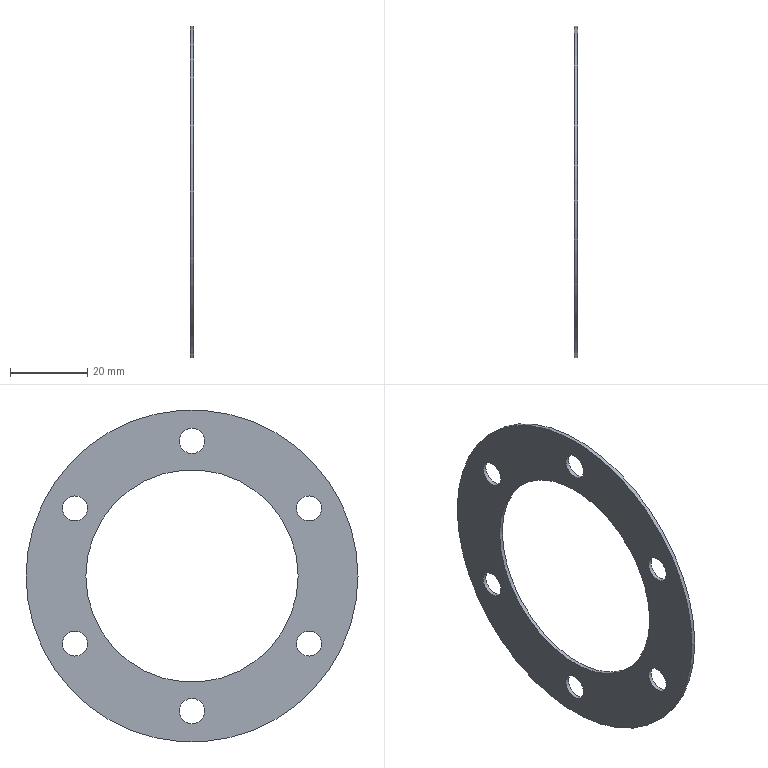Component | NX | XIAODIANPIAN_2 | 1 solid | 10 faces | box 1 x 86 x 86 mm | volume 3234 mm3 | cylinder 8 | plane 2 | commonest cylinder face diameters 6.5 x6 86 x1 55 x1
STEP:
#1=CARTESIAN_POINT('',(0.,0.,0.));
#2=DIRECTION('',(0.,0.,1.));
#3=DIRECTION('',(1.,0.,0.));
#4=AXIS2_PLACEMENT_3D('',#1,#2,#3);
#5=CARTESIAN_POINT('',(-111.,44.5,-88.));
#6=VERTEX_POINT('',#5);
#7=CARTESIAN_POINT('',(-111.,87.5,-88.));
#8=DIRECTION('',(-1.,0.,0.));
#9=DIRECTION('',(0.,-1.,0.));
#10=AXIS2_PLACEMENT_3D('',#7,#8,#9);
#11=CIRCLE('',#10,43.);
#12=CARTESIAN_POINT('',(-111.,87.5,-88.));
#13=DIRECTION('',(1.,0.,0.));
#14=DIRECTION('',(0.,0.,1.));
#15=AXIS2_PLACEMENT_3D('',#12,#13,#14);
#16=CYLINDRICAL_SURFACE('',#15,43.);
#17=CARTESIAN_POINT('',(7.854,0.));
#18=DIRECTION('',(-1.,0.));
#19=VECTOR('',#18,1.);
#20=LINE('',#17,#19);
#21=(GEOMETRIC_REPRESENTATION_CONTEXT(2)PARAMETRIC_REPRESENTATION_CONTEXT()REPRESENTATION_CONTEXT('',''));
#22=DEFINITIONAL_REPRESENTATION('',(#20),#21);
#23=PCURVE('',#16,#22);
#24=CARTESIAN_POINT('',(-111.,87.5,-88.));
#25=DIRECTION('',(-1.,0.,0.));
#26=DIRECTION('',(0.,0.,-1.));
#27=AXIS2_PLACEMENT_3D('',#24,#25,#26);
#28=PLANE('',#27);
#29=CARTESIAN_POINT('',(0.,0.));
#30=DIRECTION('',(0.,1.));
#31=AXIS2_PLACEMENT_2D('',#29,#30);
#32=CIRCLE('',#31,43.);
#33=(GEOMETRIC_REPRESENTATION_CONTEXT(2)PARAMETRIC_REPRESENTATION_CONTEXT()REPRESENTATION_CONTEXT('',''));
#34=DEFINITIONAL_REPRESENTATION('',(#32),#33);
#35=PCURVE('',#28,#34);
#36=SURFACE_CURVE('',#11,(#23,#35),.PCURVE_S1.);
#37=EDGE_CURVE('',#6,#6,#36,.T.);
#38=ORIENTED_EDGE('',*,*,#37,.F.);
#39=CARTESIAN_POINT('',(-110.,44.5,-88.));
#40=VERTEX_POINT('',#39);
#41=CARTESIAN_POINT('',(-111.,44.5,-88.));
#42=CARTESIAN_POINT('',(-110.,44.5,-88.));
#43=B_SPLINE_CURVE_WITH_KNOTS('',1,(#41,#42),.UNSPECIFIED.,.F.,.F.,(2,2),(0.,1.),.PIECEWISE_BEZIER_KNOTS.);
#44=CARTESIAN_POINT('',(7.854,0.));
#45=DIRECTION('',(0.,1.));
#46=VECTOR('',#45,1.);
#47=LINE('',#44,#46);
#48=(GEOMETRIC_REPRESENTATION_CONTEXT(2)PARAMETRIC_REPRESENTATION_CONTEXT()REPRESENTATION_CONTEXT('',''));
#49=DEFINITIONAL_REPRESENTATION('',(#47),#48);
#50=PCURVE('',#16,#49);
#51=CARTESIAN_POINT('',(1.571,0.));
#52=DIRECTION('',(0.,1.));
#53=VECTOR('',#52,1.);
#54=LINE('',#51,#53);
#55=(GEOMETRIC_REPRESENTATION_CONTEXT(2)PARAMETRIC_REPRESENTATION_CONTEXT()REPRESENTATION_CONTEXT('',''));
#56=DEFINITIONAL_REPRESENTATION('',(#54),#55);
#57=PCURVE('',#16,#56);
#58=SEAM_CURVE('',#43,(#50,#57),.PCURVE_S1.);
#59=EDGE_CURVE('',#6,#40,#58,.T.);
#60=ORIENTED_EDGE('',*,*,#59,.T.);
#61=CARTESIAN_POINT('',(-110.,87.5,-88.));
#62=DIRECTION('',(-1.,0.,0.));
#63=DIRECTION('',(0.,-1.,0.));
#64=AXIS2_PLACEMENT_3D('',#61,#62,#63);
#65=CIRCLE('',#64,43.);
#66=CARTESIAN_POINT('',(7.854,1.));
#67=DIRECTION('',(-1.,0.));
#68=VECTOR('',#67,1.);
#69=LINE('',#66,#68);
#70=(GEOMETRIC_REPRESENTATION_CONTEXT(2)PARAMETRIC_REPRESENTATION_CONTEXT()REPRESENTATION_CONTEXT('',''));
#71=DEFINITIONAL_REPRESENTATION('',(#69),#70);
#72=PCURVE('',#16,#71);
#73=CARTESIAN_POINT('',(-110.,87.5,-88.));
#74=DIRECTION('',(-1.,0.,0.));
#75=DIRECTION('',(0.,0.,-1.));
#76=AXIS2_PLACEMENT_3D('',#73,#74,#75);
#77=PLANE('',#76);
#78=CARTESIAN_POINT('',(0.,0.));
#79=DIRECTION('',(0.,1.));
#80=AXIS2_PLACEMENT_2D('',#78,#79);
#81=CIRCLE('',#80,43.);
#82=(GEOMETRIC_REPRESENTATION_CONTEXT(2)PARAMETRIC_REPRESENTATION_CONTEXT()REPRESENTATION_CONTEXT('',''));
#83=DEFINITIONAL_REPRESENTATION('',(#81),#82);
#84=PCURVE('',#77,#83);
#85=SURFACE_CURVE('',#65,(#72,#84),.PCURVE_S1.);
#86=EDGE_CURVE('',#40,#40,#85,.T.);
#87=ORIENTED_EDGE('',*,*,#86,.T.);
#88=ORIENTED_EDGE('',*,*,#59,.F.);
#89=EDGE_LOOP('',(#38,#60,#87,#88));
#90=FACE_BOUND('',#89,.T.);
#91=ADVANCED_FACE('',(#90),#16,.T.);
#92=CARTESIAN_POINT('',(-111.,60.,-88.));
#93=VERTEX_POINT('',#92);
#94=CARTESIAN_POINT('',(-111.,87.5,-88.));
#95=DIRECTION('',(-1.,0.,0.));
#96=DIRECTION('',(0.,-1.,0.));
#97=AXIS2_PLACEMENT_3D('',#94,#95,#96);
#98=CIRCLE('',#97,27.5);
#99=CARTESIAN_POINT('',(-111.,87.5,-88.));
#100=DIRECTION('',(1.,0.,0.));
#101=DIRECTION('',(0.,0.,1.));
#102=AXIS2_PLACEMENT_3D('',#99,#100,#101);
#103=CYLINDRICAL_SURFACE('',#102,27.5);
#104=CARTESIAN_POINT('',(7.854,0.));
#105=DIRECTION('',(-1.,0.));
#106=VECTOR('',#105,1.);
#107=LINE('',#104,#106);
#108=(GEOMETRIC_REPRESENTATION_CONTEXT(2)PARAMETRIC_REPRESENTATION_CONTEXT()REPRESENTATION_CONTEXT('',''));
#109=DEFINITIONAL_REPRESENTATION('',(#107),#108);
#110=PCURVE('',#103,#109);
#111=CARTESIAN_POINT('',(0.,0.));
#112=DIRECTION('',(0.,1.));
#113=AXIS2_PLACEMENT_2D('',#111,#112);
#114=CIRCLE('',#113,27.5);
#115=(GEOMETRIC_REPRESENTATION_CONTEXT(2)PARAMETRIC_REPRESENTATION_CONTEXT()REPRESENTATION_CONTEXT('',''));
#116=DEFINITIONAL_REPRESENTATION('',(#114),#115);
#117=PCURVE('',#28,#116);
#118=SURFACE_CURVE('',#98,(#110,#117),.PCURVE_S1.);
#119=EDGE_CURVE('',#93,#93,#118,.T.);
#120=ORIENTED_EDGE('',*,*,#119,.F.);
#121=CARTESIAN_POINT('',(-110.,60.,-88.));
#122=VERTEX_POINT('',#121);
#123=CARTESIAN_POINT('',(-111.,60.,-88.));
#124=CARTESIAN_POINT('',(-110.,60.,-88.));
#125=B_SPLINE_CURVE_WITH_KNOTS('',1,(#123,#124),.UNSPECIFIED.,.F.,.F.,(2,2),(0.,1.),.PIECEWISE_BEZIER_KNOTS.);
#126=CARTESIAN_POINT('',(7.854,0.));
#127=DIRECTION('',(0.,1.));
#128=VECTOR('',#127,1.);
#129=LINE('',#126,#128);
#130=(GEOMETRIC_REPRESENTATION_CONTEXT(2)PARAMETRIC_REPRESENTATION_CONTEXT()REPRESENTATION_CONTEXT('',''));
#131=DEFINITIONAL_REPRESENTATION('',(#129),#130);
#132=PCURVE('',#103,#131);
#133=CARTESIAN_POINT('',(1.571,0.));
#134=DIRECTION('',(0.,1.));
#135=VECTOR('',#134,1.);
#136=LINE('',#133,#135);
#137=(GEOMETRIC_REPRESENTATION_CONTEXT(2)PARAMETRIC_REPRESENTATION_CONTEXT()REPRESENTATION_CONTEXT('',''));
#138=DEFINITIONAL_REPRESENTATION('',(#136),#137);
#139=PCURVE('',#103,#138);
#140=SEAM_CURVE('',#125,(#132,#139),.PCURVE_S1.);
#141=EDGE_CURVE('',#93,#122,#140,.T.);
#142=ORIENTED_EDGE('',*,*,#141,.T.);
#143=CARTESIAN_POINT('',(-110.,87.5,-88.));
#144=DIRECTION('',(-1.,0.,0.));
#145=DIRECTION('',(0.,-1.,0.));
#146=AXIS2_PLACEMENT_3D('',#143,#144,#145);
#147=CIRCLE('',#146,27.5);
#148=CARTESIAN_POINT('',(7.854,1.));
#149=DIRECTION('',(-1.,0.));
#150=VECTOR('',#149,1.);
#151=LINE('',#148,#150);
#152=(GEOMETRIC_REPRESENTATION_CONTEXT(2)PARAMETRIC_REPRESENTATION_CONTEXT()REPRESENTATION_CONTEXT('',''));
#153=DEFINITIONAL_REPRESENTATION('',(#151),#152);
#154=PCURVE('',#103,#153);
#155=CARTESIAN_POINT('',(0.,0.));
#156=DIRECTION('',(0.,1.));
#157=AXIS2_PLACEMENT_2D('',#155,#156);
#158=CIRCLE('',#157,27.5);
#159=(GEOMETRIC_REPRESENTATION_CONTEXT(2)PARAMETRIC_REPRESENTATION_CONTEXT()REPRESENTATION_CONTEXT('',''));
#160=DEFINITIONAL_REPRESENTATION('',(#158),#159);
#161=PCURVE('',#77,#160);
#162=SURFACE_CURVE('',#147,(#154,#161),.PCURVE_S1.);
#163=EDGE_CURVE('',#122,#122,#162,.T.);
#164=ORIENTED_EDGE('',*,*,#163,.T.);
#165=ORIENTED_EDGE('',*,*,#141,.F.);
#166=EDGE_LOOP('',(#120,#142,#164,#165));
#167=FACE_BOUND('',#166,.F.);
#168=ADVANCED_FACE('',(#167),#103,.F.);
#169=CARTESIAN_POINT('',(-111.,57.189,-73.75));
#170=VERTEX_POINT('',#169);
#171=CARTESIAN_POINT('',(-111.,57.189,-70.5));
#172=DIRECTION('',(-1.,0.,0.));
#173=DIRECTION('',(0.,0.,-1.));
#174=AXIS2_PLACEMENT_3D('',#171,#172,#173);
#175=CIRCLE('',#174,3.25);
#176=CARTESIAN_POINT('',(-17.5,30.311));
#177=DIRECTION('',(1.,0.));
#178=AXIS2_PLACEMENT_2D('',#176,#177);
#179=CIRCLE('',#178,3.25);
#180=(GEOMETRIC_REPRESENTATION_CONTEXT(2)PARAMETRIC_REPRESENTATION_CONTEXT()REPRESENTATION_CONTEXT('',''));
#181=DEFINITIONAL_REPRESENTATION('',(#179),#180);
#182=PCURVE('',#28,#181);
#183=CARTESIAN_POINT('',(-110.,57.189,-70.5));
#184=DIRECTION('',(-1.,0.,0.));
#185=DIRECTION('',(0.,0.,-1.));
#186=AXIS2_PLACEMENT_3D('',#183,#184,#185);
#187=CYLINDRICAL_SURFACE('',#186,3.25);
#188=CARTESIAN_POINT('',(0.,1.));
#189=DIRECTION('',(1.,0.));
#190=VECTOR('',#189,1.);
#191=LINE('',#188,#190);
#192=(GEOMETRIC_REPRESENTATION_CONTEXT(2)PARAMETRIC_REPRESENTATION_CONTEXT()REPRESENTATION_CONTEXT('',''));
#193=DEFINITIONAL_REPRESENTATION('',(#191),#192);
#194=PCURVE('',#187,#193);
#195=SURFACE_CURVE('',#175,(#182,#194),.PCURVE_S1.);
#196=EDGE_CURVE('',#170,#170,#195,.T.);
#197=ORIENTED_EDGE('',*,*,#196,.F.);
#198=EDGE_LOOP('',(#197));
#199=FACE_BOUND('',#198,.T.);
#200=CARTESIAN_POINT('',(-111.,57.189,-108.75));
#201=VERTEX_POINT('',#200);
#202=CARTESIAN_POINT('',(-111.,57.189,-105.5));
#203=DIRECTION('',(-1.,0.,0.));
#204=DIRECTION('',(0.,0.,-1.));
#205=AXIS2_PLACEMENT_3D('',#202,#203,#204);
#206=CIRCLE('',#205,3.25);
#207=CARTESIAN_POINT('',(17.5,30.311));
#208=DIRECTION('',(1.,0.));
#209=AXIS2_PLACEMENT_2D('',#207,#208);
#210=CIRCLE('',#209,3.25);
#211=(GEOMETRIC_REPRESENTATION_CONTEXT(2)PARAMETRIC_REPRESENTATION_CONTEXT()REPRESENTATION_CONTEXT('',''));
#212=DEFINITIONAL_REPRESENTATION('',(#210),#211);
#213=PCURVE('',#28,#212);
#214=CARTESIAN_POINT('',(-110.,57.189,-105.5));
#215=DIRECTION('',(-1.,0.,0.));
#216=DIRECTION('',(0.,0.,-1.));
#217=AXIS2_PLACEMENT_3D('',#214,#215,#216);
#218=CYLINDRICAL_SURFACE('',#217,3.25);
#219=CARTESIAN_POINT('',(0.,1.));
#220=DIRECTION('',(1.,0.));
#221=VECTOR('',#220,1.);
#222=LINE('',#219,#221);
#223=(GEOMETRIC_REPRESENTATION_CONTEXT(2)PARAMETRIC_REPRESENTATION_CONTEXT()REPRESENTATION_CONTEXT('',''));
#224=DEFINITIONAL_REPRESENTATION('',(#222),#223);
#225=PCURVE('',#218,#224);
#226=SURFACE_CURVE('',#206,(#213,#225),.PCURVE_S1.);
#227=EDGE_CURVE('',#201,#201,#226,.T.);
#228=ORIENTED_EDGE('',*,*,#227,.F.);
#229=EDGE_LOOP('',(#228));
#230=FACE_BOUND('',#229,.T.);
#231=CARTESIAN_POINT('',(-111.,87.5,-56.25));
#232=VERTEX_POINT('',#231);
#233=CARTESIAN_POINT('',(-111.,87.5,-53.));
#234=DIRECTION('',(-1.,0.,0.));
#235=DIRECTION('',(0.,0.,-1.));
#236=AXIS2_PLACEMENT_3D('',#233,#234,#235);
#237=CIRCLE('',#236,3.25);
#238=CARTESIAN_POINT('',(-35.,-0.));
#239=DIRECTION('',(1.,0.));
#240=AXIS2_PLACEMENT_2D('',#238,#239);
#241=CIRCLE('',#240,3.25);
#242=(GEOMETRIC_REPRESENTATION_CONTEXT(2)PARAMETRIC_REPRESENTATION_CONTEXT()REPRESENTATION_CONTEXT('',''));
#243=DEFINITIONAL_REPRESENTATION('',(#241),#242);
#244=PCURVE('',#28,#243);
#245=CARTESIAN_POINT('',(-110.,87.5,-53.));
#246=DIRECTION('',(-1.,0.,0.));
#247=DIRECTION('',(0.,0.,-1.));
#248=AXIS2_PLACEMENT_3D('',#245,#246,#247);
#249=CYLINDRICAL_SURFACE('',#248,3.25);
#250=CARTESIAN_POINT('',(0.,1.));
#251=DIRECTION('',(1.,0.));
#252=VECTOR('',#251,1.);
#253=LINE('',#250,#252);
#254=(GEOMETRIC_REPRESENTATION_CONTEXT(2)PARAMETRIC_REPRESENTATION_CONTEXT()REPRESENTATION_CONTEXT('',''));
#255=DEFINITIONAL_REPRESENTATION('',(#253),#254);
#256=PCURVE('',#249,#255);
#257=SURFACE_CURVE('',#237,(#244,#256),.PCURVE_S1.);
#258=EDGE_CURVE('',#232,#232,#257,.T.);
#259=ORIENTED_EDGE('',*,*,#258,.F.);
#260=EDGE_LOOP('',(#259));
#261=FACE_BOUND('',#260,.T.);
#262=CARTESIAN_POINT('',(-111.,87.5,-126.25));
#263=VERTEX_POINT('',#262);
#264=CARTESIAN_POINT('',(-111.,87.5,-123.));
#265=DIRECTION('',(-1.,0.,0.));
#266=DIRECTION('',(0.,0.,-1.));
#267=AXIS2_PLACEMENT_3D('',#264,#265,#266);
#268=CIRCLE('',#267,3.25);
#269=CARTESIAN_POINT('',(35.,0.));
#270=DIRECTION('',(1.,0.));
#271=AXIS2_PLACEMENT_2D('',#269,#270);
#272=CIRCLE('',#271,3.25);
#273=(GEOMETRIC_REPRESENTATION_CONTEXT(2)PARAMETRIC_REPRESENTATION_CONTEXT()REPRESENTATION_CONTEXT('',''));
#274=DEFINITIONAL_REPRESENTATION('',(#272),#273);
#275=PCURVE('',#28,#274);
#276=CARTESIAN_POINT('',(-110.,87.5,-123.));
#277=DIRECTION('',(-1.,0.,0.));
#278=DIRECTION('',(0.,0.,-1.));
#279=AXIS2_PLACEMENT_3D('',#276,#277,#278);
#280=CYLINDRICAL_SURFACE('',#279,3.25);
#281=CARTESIAN_POINT('',(0.,1.));
#282=DIRECTION('',(1.,0.));
#283=VECTOR('',#282,1.);
#284=LINE('',#281,#283);
#285=(GEOMETRIC_REPRESENTATION_CONTEXT(2)PARAMETRIC_REPRESENTATION_CONTEXT()REPRESENTATION_CONTEXT('',''));
#286=DEFINITIONAL_REPRESENTATION('',(#284),#285);
#287=PCURVE('',#280,#286);
#288=SURFACE_CURVE('',#268,(#275,#287),.PCURVE_S1.);
#289=EDGE_CURVE('',#263,#263,#288,.T.);
#290=ORIENTED_EDGE('',*,*,#289,.F.);
#291=EDGE_LOOP('',(#290));
#292=FACE_BOUND('',#291,.T.);
#293=CARTESIAN_POINT('',(-111.,117.811,-73.75));
#294=VERTEX_POINT('',#293);
#295=CARTESIAN_POINT('',(-111.,117.811,-70.5));
#296=DIRECTION('',(-1.,0.,0.));
#297=DIRECTION('',(0.,0.,-1.));
#298=AXIS2_PLACEMENT_3D('',#295,#296,#297);
#299=CIRCLE('',#298,3.25);
#300=CARTESIAN_POINT('',(-17.5,-30.311));
#301=DIRECTION('',(1.,0.));
#302=AXIS2_PLACEMENT_2D('',#300,#301);
#303=CIRCLE('',#302,3.25);
#304=(GEOMETRIC_REPRESENTATION_CONTEXT(2)PARAMETRIC_REPRESENTATION_CONTEXT()REPRESENTATION_CONTEXT('',''));
#305=DEFINITIONAL_REPRESENTATION('',(#303),#304);
#306=PCURVE('',#28,#305);
#307=CARTESIAN_POINT('',(-110.,117.811,-70.5));
#308=DIRECTION('',(-1.,0.,0.));
#309=DIRECTION('',(0.,0.,-1.));
#310=AXIS2_PLACEMENT_3D('',#307,#308,#309);
#311=CYLINDRICAL_SURFACE('',#310,3.25);
#312=CARTESIAN_POINT('',(0.,1.));
#313=DIRECTION('',(1.,0.));
#314=VECTOR('',#313,1.);
#315=LINE('',#312,#314);
#316=(GEOMETRIC_REPRESENTATION_CONTEXT(2)PARAMETRIC_REPRESENTATION_CONTEXT()REPRESENTATION_CONTEXT('',''));
#317=DEFINITIONAL_REPRESENTATION('',(#315),#316);
#318=PCURVE('',#311,#317);
#319=SURFACE_CURVE('',#299,(#306,#318),.PCURVE_S1.);
#320=EDGE_CURVE('',#294,#294,#319,.T.);
#321=ORIENTED_EDGE('',*,*,#320,.F.);
#322=EDGE_LOOP('',(#321));
#323=FACE_BOUND('',#322,.T.);
#324=CARTESIAN_POINT('',(-111.,117.811,-108.75));
#325=VERTEX_POINT('',#324);
#326=CARTESIAN_POINT('',(-111.,117.811,-105.5));
#327=DIRECTION('',(-1.,0.,0.));
#328=DIRECTION('',(0.,0.,-1.));
#329=AXIS2_PLACEMENT_3D('',#326,#327,#328);
#330=CIRCLE('',#329,3.25);
#331=CARTESIAN_POINT('',(17.5,-30.311));
#332=DIRECTION('',(1.,0.));
#333=AXIS2_PLACEMENT_2D('',#331,#332);
#334=CIRCLE('',#333,3.25);
#335=(GEOMETRIC_REPRESENTATION_CONTEXT(2)PARAMETRIC_REPRESENTATION_CONTEXT()REPRESENTATION_CONTEXT('',''));
#336=DEFINITIONAL_REPRESENTATION('',(#334),#335);
#337=PCURVE('',#28,#336);
#338=CARTESIAN_POINT('',(-110.,117.811,-105.5));
#339=DIRECTION('',(-1.,0.,0.));
#340=DIRECTION('',(0.,0.,-1.));
#341=AXIS2_PLACEMENT_3D('',#338,#339,#340);
#342=CYLINDRICAL_SURFACE('',#341,3.25);
#343=CARTESIAN_POINT('',(0.,1.));
#344=DIRECTION('',(1.,0.));
#345=VECTOR('',#344,1.);
#346=LINE('',#343,#345);
#347=(GEOMETRIC_REPRESENTATION_CONTEXT(2)PARAMETRIC_REPRESENTATION_CONTEXT()REPRESENTATION_CONTEXT('',''));
#348=DEFINITIONAL_REPRESENTATION('',(#346),#347);
#349=PCURVE('',#342,#348);
#350=SURFACE_CURVE('',#330,(#337,#349),.PCURVE_S1.);
#351=EDGE_CURVE('',#325,#325,#350,.T.);
#352=ORIENTED_EDGE('',*,*,#351,.F.);
#353=EDGE_LOOP('',(#352));
#354=FACE_BOUND('',#353,.T.);
#355=ORIENTED_EDGE('',*,*,#37,.T.);
#356=EDGE_LOOP('',(#355));
#357=FACE_BOUND('',#356,.T.);
#358=ORIENTED_EDGE('',*,*,#119,.F.);
#359=EDGE_LOOP('',(#358));
#360=FACE_BOUND('',#359,.T.);
#361=ADVANCED_FACE('',(#199,#230,#261,#292,#323,#354,#357,#360),#28,.T.);
#362=CARTESIAN_POINT('',(-110.,57.189,-73.75));
#363=VERTEX_POINT('',#362);
#364=CARTESIAN_POINT('',(-110.,57.189,-70.5));
#365=DIRECTION('',(-1.,0.,0.));
#366=DIRECTION('',(0.,0.,-1.));
#367=AXIS2_PLACEMENT_3D('',#364,#365,#366);
#368=CIRCLE('',#367,3.25);
#369=CARTESIAN_POINT('',(-17.5,30.311));
#370=DIRECTION('',(1.,0.));
#371=AXIS2_PLACEMENT_2D('',#369,#370);
#372=CIRCLE('',#371,3.25);
#373=(GEOMETRIC_REPRESENTATION_CONTEXT(2)PARAMETRIC_REPRESENTATION_CONTEXT()REPRESENTATION_CONTEXT('',''));
#374=DEFINITIONAL_REPRESENTATION('',(#372),#373);
#375=PCURVE('',#77,#374);
#376=CARTESIAN_POINT('',(0.,0.));
#377=DIRECTION('',(1.,0.));
#378=VECTOR('',#377,1.);
#379=LINE('',#376,#378);
#380=(GEOMETRIC_REPRESENTATION_CONTEXT(2)PARAMETRIC_REPRESENTATION_CONTEXT()REPRESENTATION_CONTEXT('',''));
#381=DEFINITIONAL_REPRESENTATION('',(#379),#380);
#382=PCURVE('',#187,#381);
#383=SURFACE_CURVE('',#368,(#375,#382),.PCURVE_S1.);
#384=EDGE_CURVE('',#363,#363,#383,.T.);
#385=ORIENTED_EDGE('',*,*,#384,.T.);
#386=EDGE_LOOP('',(#385));
#387=FACE_BOUND('',#386,.T.);
#388=CARTESIAN_POINT('',(-110.,57.189,-108.75));
#389=VERTEX_POINT('',#388);
#390=CARTESIAN_POINT('',(-110.,57.189,-105.5));
#391=DIRECTION('',(-1.,0.,0.));
#392=DIRECTION('',(0.,0.,-1.));
#393=AXIS2_PLACEMENT_3D('',#390,#391,#392);
#394=CIRCLE('',#393,3.25);
#395=CARTESIAN_POINT('',(17.5,30.311));
#396=DIRECTION('',(1.,0.));
#397=AXIS2_PLACEMENT_2D('',#395,#396);
#398=CIRCLE('',#397,3.25);
#399=(GEOMETRIC_REPRESENTATION_CONTEXT(2)PARAMETRIC_REPRESENTATION_CONTEXT()REPRESENTATION_CONTEXT('',''));
#400=DEFINITIONAL_REPRESENTATION('',(#398),#399);
#401=PCURVE('',#77,#400);
#402=CARTESIAN_POINT('',(0.,0.));
#403=DIRECTION('',(1.,0.));
#404=VECTOR('',#403,1.);
#405=LINE('',#402,#404);
#406=(GEOMETRIC_REPRESENTATION_CONTEXT(2)PARAMETRIC_REPRESENTATION_CONTEXT()REPRESENTATION_CONTEXT('',''));
#407=DEFINITIONAL_REPRESENTATION('',(#405),#406);
#408=PCURVE('',#218,#407);
#409=SURFACE_CURVE('',#394,(#401,#408),.PCURVE_S1.);
#410=EDGE_CURVE('',#389,#389,#409,.T.);
#411=ORIENTED_EDGE('',*,*,#410,.T.);
#412=EDGE_LOOP('',(#411));
#413=FACE_BOUND('',#412,.T.);
#414=CARTESIAN_POINT('',(-110.,87.5,-56.25));
#415=VERTEX_POINT('',#414);
#416=CARTESIAN_POINT('',(-110.,87.5,-53.));
#417=DIRECTION('',(-1.,0.,0.));
#418=DIRECTION('',(0.,0.,-1.));
#419=AXIS2_PLACEMENT_3D('',#416,#417,#418);
#420=CIRCLE('',#419,3.25);
#421=CARTESIAN_POINT('',(-35.,-0.));
#422=DIRECTION('',(1.,0.));
#423=AXIS2_PLACEMENT_2D('',#421,#422);
#424=CIRCLE('',#423,3.25);
#425=(GEOMETRIC_REPRESENTATION_CONTEXT(2)PARAMETRIC_REPRESENTATION_CONTEXT()REPRESENTATION_CONTEXT('',''));
#426=DEFINITIONAL_REPRESENTATION('',(#424),#425);
#427=PCURVE('',#77,#426);
#428=CARTESIAN_POINT('',(0.,0.));
#429=DIRECTION('',(1.,0.));
#430=VECTOR('',#429,1.);
#431=LINE('',#428,#430);
#432=(GEOMETRIC_REPRESENTATION_CONTEXT(2)PARAMETRIC_REPRESENTATION_CONTEXT()REPRESENTATION_CONTEXT('',''));
#433=DEFINITIONAL_REPRESENTATION('',(#431),#432);
#434=PCURVE('',#249,#433);
#435=SURFACE_CURVE('',#420,(#427,#434),.PCURVE_S1.);
#436=EDGE_CURVE('',#415,#415,#435,.T.);
#437=ORIENTED_EDGE('',*,*,#436,.T.);
#438=EDGE_LOOP('',(#437));
#439=FACE_BOUND('',#438,.T.);
#440=CARTESIAN_POINT('',(-110.,87.5,-126.25));
#441=VERTEX_POINT('',#440);
#442=CARTESIAN_POINT('',(-110.,87.5,-123.));
#443=DIRECTION('',(-1.,0.,0.));
#444=DIRECTION('',(0.,0.,-1.));
#445=AXIS2_PLACEMENT_3D('',#442,#443,#444);
#446=CIRCLE('',#445,3.25);
#447=CARTESIAN_POINT('',(35.,0.));
#448=DIRECTION('',(1.,0.));
#449=AXIS2_PLACEMENT_2D('',#447,#448);
#450=CIRCLE('',#449,3.25);
#451=(GEOMETRIC_REPRESENTATION_CONTEXT(2)PARAMETRIC_REPRESENTATION_CONTEXT()REPRESENTATION_CONTEXT('',''));
#452=DEFINITIONAL_REPRESENTATION('',(#450),#451);
#453=PCURVE('',#77,#452);
#454=CARTESIAN_POINT('',(0.,0.));
#455=DIRECTION('',(1.,0.));
#456=VECTOR('',#455,1.);
#457=LINE('',#454,#456);
#458=(GEOMETRIC_REPRESENTATION_CONTEXT(2)PARAMETRIC_REPRESENTATION_CONTEXT()REPRESENTATION_CONTEXT('',''));
#459=DEFINITIONAL_REPRESENTATION('',(#457),#458);
#460=PCURVE('',#280,#459);
#461=SURFACE_CURVE('',#446,(#453,#460),.PCURVE_S1.);
#462=EDGE_CURVE('',#441,#441,#461,.T.);
#463=ORIENTED_EDGE('',*,*,#462,.T.);
#464=EDGE_LOOP('',(#463));
#465=FACE_BOUND('',#464,.T.);
#466=CARTESIAN_POINT('',(-110.,117.811,-73.75));
#467=VERTEX_POINT('',#466);
#468=CARTESIAN_POINT('',(-110.,117.811,-70.5));
#469=DIRECTION('',(-1.,0.,0.));
#470=DIRECTION('',(0.,0.,-1.));
#471=AXIS2_PLACEMENT_3D('',#468,#469,#470);
#472=CIRCLE('',#471,3.25);
#473=CARTESIAN_POINT('',(-17.5,-30.311));
#474=DIRECTION('',(1.,0.));
#475=AXIS2_PLACEMENT_2D('',#473,#474);
#476=CIRCLE('',#475,3.25);
#477=(GEOMETRIC_REPRESENTATION_CONTEXT(2)PARAMETRIC_REPRESENTATION_CONTEXT()REPRESENTATION_CONTEXT('',''));
#478=DEFINITIONAL_REPRESENTATION('',(#476),#477);
#479=PCURVE('',#77,#478);
#480=CARTESIAN_POINT('',(0.,0.));
#481=DIRECTION('',(1.,0.));
#482=VECTOR('',#481,1.);
#483=LINE('',#480,#482);
#484=(GEOMETRIC_REPRESENTATION_CONTEXT(2)PARAMETRIC_REPRESENTATION_CONTEXT()REPRESENTATION_CONTEXT('',''));
#485=DEFINITIONAL_REPRESENTATION('',(#483),#484);
#486=PCURVE('',#311,#485);
#487=SURFACE_CURVE('',#472,(#479,#486),.PCURVE_S1.);
#488=EDGE_CURVE('',#467,#467,#487,.T.);
#489=ORIENTED_EDGE('',*,*,#488,.T.);
#490=EDGE_LOOP('',(#489));
#491=FACE_BOUND('',#490,.T.);
#492=CARTESIAN_POINT('',(-110.,117.811,-108.75));
#493=VERTEX_POINT('',#492);
#494=CARTESIAN_POINT('',(-110.,117.811,-105.5));
#495=DIRECTION('',(-1.,0.,0.));
#496=DIRECTION('',(0.,0.,-1.));
#497=AXIS2_PLACEMENT_3D('',#494,#495,#496);
#498=CIRCLE('',#497,3.25);
#499=CARTESIAN_POINT('',(17.5,-30.311));
#500=DIRECTION('',(1.,0.));
#501=AXIS2_PLACEMENT_2D('',#499,#500);
#502=CIRCLE('',#501,3.25);
#503=(GEOMETRIC_REPRESENTATION_CONTEXT(2)PARAMETRIC_REPRESENTATION_CONTEXT()REPRESENTATION_CONTEXT('',''));
#504=DEFINITIONAL_REPRESENTATION('',(#502),#503);
#505=PCURVE('',#77,#504);
#506=CARTESIAN_POINT('',(0.,0.));
#507=DIRECTION('',(1.,0.));
#508=VECTOR('',#507,1.);
#509=LINE('',#506,#508);
#510=(GEOMETRIC_REPRESENTATION_CONTEXT(2)PARAMETRIC_REPRESENTATION_CONTEXT()REPRESENTATION_CONTEXT('',''));
#511=DEFINITIONAL_REPRESENTATION('',(#509),#510);
#512=PCURVE('',#342,#511);
#513=SURFACE_CURVE('',#498,(#505,#512),.PCURVE_S1.);
#514=EDGE_CURVE('',#493,#493,#513,.T.);
#515=ORIENTED_EDGE('',*,*,#514,.T.);
#516=EDGE_LOOP('',(#515));
#517=FACE_BOUND('',#516,.T.);
#518=ORIENTED_EDGE('',*,*,#86,.F.);
#519=EDGE_LOOP('',(#518));
#520=FACE_BOUND('',#519,.T.);
#521=ORIENTED_EDGE('',*,*,#163,.T.);
#522=EDGE_LOOP('',(#521));
#523=FACE_BOUND('',#522,.T.);
#524=ADVANCED_FACE('',(#387,#413,#439,#465,#491,#517,#520,#523),#77,.F.);
#525=ORIENTED_EDGE('',*,*,#351,.F.);
#526=CARTESIAN_POINT('',(-110.,117.811,-108.75));
#527=CARTESIAN_POINT('',(-111.,117.811,-108.75));
#528=B_SPLINE_CURVE_WITH_KNOTS('',1,(#526,#527),.UNSPECIFIED.,.F.,.F.,(2,2),(0.,1.),.PIECEWISE_BEZIER_KNOTS.);
#529=CARTESIAN_POINT('',(0.,0.));
#530=DIRECTION('',(0.,1.));
#531=VECTOR('',#530,1.);
#532=LINE('',#529,#531);
#533=(GEOMETRIC_REPRESENTATION_CONTEXT(2)PARAMETRIC_REPRESENTATION_CONTEXT()REPRESENTATION_CONTEXT('',''));
#534=DEFINITIONAL_REPRESENTATION('',(#532),#533);
#535=PCURVE('',#342,#534);
#536=CARTESIAN_POINT('',(6.283,0.));
#537=DIRECTION('',(0.,1.));
#538=VECTOR('',#537,1.);
#539=LINE('',#536,#538);
#540=(GEOMETRIC_REPRESENTATION_CONTEXT(2)PARAMETRIC_REPRESENTATION_CONTEXT()REPRESENTATION_CONTEXT('',''));
#541=DEFINITIONAL_REPRESENTATION('',(#539),#540);
#542=PCURVE('',#342,#541);
#543=SEAM_CURVE('',#528,(#535,#542),.PCURVE_S1.);
#544=EDGE_CURVE('',#493,#325,#543,.T.);
#545=ORIENTED_EDGE('',*,*,#544,.F.);
#546=ORIENTED_EDGE('',*,*,#514,.T.);
#547=ORIENTED_EDGE('',*,*,#544,.T.);
#548=EDGE_LOOP('',(#525,#545,#546,#547));
#549=FACE_BOUND('',#548,.F.);
#550=ADVANCED_FACE('',(#549),#342,.F.);
#551=ORIENTED_EDGE('',*,*,#320,.F.);
#552=CARTESIAN_POINT('',(-110.,117.811,-73.75));
#553=CARTESIAN_POINT('',(-111.,117.811,-73.75));
#554=B_SPLINE_CURVE_WITH_KNOTS('',1,(#552,#553),.UNSPECIFIED.,.F.,.F.,(2,2),(0.,1.),.PIECEWISE_BEZIER_KNOTS.);
#555=CARTESIAN_POINT('',(0.,0.));
#556=DIRECTION('',(0.,1.));
#557=VECTOR('',#556,1.);
#558=LINE('',#555,#557);
#559=(GEOMETRIC_REPRESENTATION_CONTEXT(2)PARAMETRIC_REPRESENTATION_CONTEXT()REPRESENTATION_CONTEXT('',''));
#560=DEFINITIONAL_REPRESENTATION('',(#558),#559);
#561=PCURVE('',#311,#560);
#562=CARTESIAN_POINT('',(6.283,0.));
#563=DIRECTION('',(0.,1.));
#564=VECTOR('',#563,1.);
#565=LINE('',#562,#564);
#566=(GEOMETRIC_REPRESENTATION_CONTEXT(2)PARAMETRIC_REPRESENTATION_CONTEXT()REPRESENTATION_CONTEXT('',''));
#567=DEFINITIONAL_REPRESENTATION('',(#565),#566);
#568=PCURVE('',#311,#567);
#569=SEAM_CURVE('',#554,(#561,#568),.PCURVE_S1.);
#570=EDGE_CURVE('',#467,#294,#569,.T.);
#571=ORIENTED_EDGE('',*,*,#570,.F.);
#572=ORIENTED_EDGE('',*,*,#488,.T.);
#573=ORIENTED_EDGE('',*,*,#570,.T.);
#574=EDGE_LOOP('',(#551,#571,#572,#573));
#575=FACE_BOUND('',#574,.F.);
#576=ADVANCED_FACE('',(#575),#311,.F.);
#577=ORIENTED_EDGE('',*,*,#289,.F.);
#578=CARTESIAN_POINT('',(-110.,87.5,-126.25));
#579=CARTESIAN_POINT('',(-111.,87.5,-126.25));
#580=B_SPLINE_CURVE_WITH_KNOTS('',1,(#578,#579),.UNSPECIFIED.,.F.,.F.,(2,2),(0.,1.),.PIECEWISE_BEZIER_KNOTS.);
#581=CARTESIAN_POINT('',(0.,0.));
#582=DIRECTION('',(0.,1.));
#583=VECTOR('',#582,1.);
#584=LINE('',#581,#583);
#585=(GEOMETRIC_REPRESENTATION_CONTEXT(2)PARAMETRIC_REPRESENTATION_CONTEXT()REPRESENTATION_CONTEXT('',''));
#586=DEFINITIONAL_REPRESENTATION('',(#584),#585);
#587=PCURVE('',#280,#586);
#588=CARTESIAN_POINT('',(6.283,0.));
#589=DIRECTION('',(0.,1.));
#590=VECTOR('',#589,1.);
#591=LINE('',#588,#590);
#592=(GEOMETRIC_REPRESENTATION_CONTEXT(2)PARAMETRIC_REPRESENTATION_CONTEXT()REPRESENTATION_CONTEXT('',''));
#593=DEFINITIONAL_REPRESENTATION('',(#591),#592);
#594=PCURVE('',#280,#593);
#595=SEAM_CURVE('',#580,(#587,#594),.PCURVE_S1.);
#596=EDGE_CURVE('',#441,#263,#595,.T.);
#597=ORIENTED_EDGE('',*,*,#596,.F.);
#598=ORIENTED_EDGE('',*,*,#462,.T.);
#599=ORIENTED_EDGE('',*,*,#596,.T.);
#600=EDGE_LOOP('',(#577,#597,#598,#599));
#601=FACE_BOUND('',#600,.F.);
#602=ADVANCED_FACE('',(#601),#280,.F.);
#603=ORIENTED_EDGE('',*,*,#258,.F.);
#604=CARTESIAN_POINT('',(-110.,87.5,-56.25));
#605=CARTESIAN_POINT('',(-111.,87.5,-56.25));
#606=B_SPLINE_CURVE_WITH_KNOTS('',1,(#604,#605),.UNSPECIFIED.,.F.,.F.,(2,2),(0.,1.),.PIECEWISE_BEZIER_KNOTS.);
#607=CARTESIAN_POINT('',(0.,0.));
#608=DIRECTION('',(0.,1.));
#609=VECTOR('',#608,1.);
#610=LINE('',#607,#609);
#611=(GEOMETRIC_REPRESENTATION_CONTEXT(2)PARAMETRIC_REPRESENTATION_CONTEXT()REPRESENTATION_CONTEXT('',''));
#612=DEFINITIONAL_REPRESENTATION('',(#610),#611);
#613=PCURVE('',#249,#612);
#614=CARTESIAN_POINT('',(6.283,0.));
#615=DIRECTION('',(0.,1.));
#616=VECTOR('',#615,1.);
#617=LINE('',#614,#616);
#618=(GEOMETRIC_REPRESENTATION_CONTEXT(2)PARAMETRIC_REPRESENTATION_CONTEXT()REPRESENTATION_CONTEXT('',''));
#619=DEFINITIONAL_REPRESENTATION('',(#617),#618);
#620=PCURVE('',#249,#619);
#621=SEAM_CURVE('',#606,(#613,#620),.PCURVE_S1.);
#622=EDGE_CURVE('',#415,#232,#621,.T.);
#623=ORIENTED_EDGE('',*,*,#622,.F.);
#624=ORIENTED_EDGE('',*,*,#436,.T.);
#625=ORIENTED_EDGE('',*,*,#622,.T.);
#626=EDGE_LOOP('',(#603,#623,#624,#625));
#627=FACE_BOUND('',#626,.F.);
#628=ADVANCED_FACE('',(#627),#249,.F.);
#629=ORIENTED_EDGE('',*,*,#227,.F.);
#630=CARTESIAN_POINT('',(-110.,57.189,-108.75));
#631=CARTESIAN_POINT('',(-111.,57.189,-108.75));
#632=B_SPLINE_CURVE_WITH_KNOTS('',1,(#630,#631),.UNSPECIFIED.,.F.,.F.,(2,2),(0.,1.),.PIECEWISE_BEZIER_KNOTS.);
#633=CARTESIAN_POINT('',(0.,0.));
#634=DIRECTION('',(0.,1.));
#635=VECTOR('',#634,1.);
#636=LINE('',#633,#635);
#637=(GEOMETRIC_REPRESENTATION_CONTEXT(2)PARAMETRIC_REPRESENTATION_CONTEXT()REPRESENTATION_CONTEXT('',''));
#638=DEFINITIONAL_REPRESENTATION('',(#636),#637);
#639=PCURVE('',#218,#638);
#640=CARTESIAN_POINT('',(6.283,0.));
#641=DIRECTION('',(0.,1.));
#642=VECTOR('',#641,1.);
#643=LINE('',#640,#642);
#644=(GEOMETRIC_REPRESENTATION_CONTEXT(2)PARAMETRIC_REPRESENTATION_CONTEXT()REPRESENTATION_CONTEXT('',''));
#645=DEFINITIONAL_REPRESENTATION('',(#643),#644);
#646=PCURVE('',#218,#645);
#647=SEAM_CURVE('',#632,(#639,#646),.PCURVE_S1.);
#648=EDGE_CURVE('',#389,#201,#647,.T.);
#649=ORIENTED_EDGE('',*,*,#648,.F.);
#650=ORIENTED_EDGE('',*,*,#410,.T.);
#651=ORIENTED_EDGE('',*,*,#648,.T.);
#652=EDGE_LOOP('',(#629,#649,#650,#651));
#653=FACE_BOUND('',#652,.F.);
#654=ADVANCED_FACE('',(#653),#218,.F.);
#655=ORIENTED_EDGE('',*,*,#196,.F.);
#656=CARTESIAN_POINT('',(-110.,57.189,-73.75));
#657=CARTESIAN_POINT('',(-111.,57.189,-73.75));
#658=B_SPLINE_CURVE_WITH_KNOTS('',1,(#656,#657),.UNSPECIFIED.,.F.,.F.,(2,2),(0.,1.),.PIECEWISE_BEZIER_KNOTS.);
#659=CARTESIAN_POINT('',(0.,0.));
#660=DIRECTION('',(0.,1.));
#661=VECTOR('',#660,1.);
#662=LINE('',#659,#661);
#663=(GEOMETRIC_REPRESENTATION_CONTEXT(2)PARAMETRIC_REPRESENTATION_CONTEXT()REPRESENTATION_CONTEXT('',''));
#664=DEFINITIONAL_REPRESENTATION('',(#662),#663);
#665=PCURVE('',#187,#664);
#666=CARTESIAN_POINT('',(6.283,0.));
#667=DIRECTION('',(0.,1.));
#668=VECTOR('',#667,1.);
#669=LINE('',#666,#668);
#670=(GEOMETRIC_REPRESENTATION_CONTEXT(2)PARAMETRIC_REPRESENTATION_CONTEXT()REPRESENTATION_CONTEXT('',''));
#671=DEFINITIONAL_REPRESENTATION('',(#669),#670);
#672=PCURVE('',#187,#671);
#673=SEAM_CURVE('',#658,(#665,#672),.PCURVE_S1.);
#674=EDGE_CURVE('',#363,#170,#673,.T.);
#675=ORIENTED_EDGE('',*,*,#674,.F.);
#676=ORIENTED_EDGE('',*,*,#384,.T.);
#677=ORIENTED_EDGE('',*,*,#674,.T.);
#678=EDGE_LOOP('',(#655,#675,#676,#677));
#679=FACE_BOUND('',#678,.F.);
#680=ADVANCED_FACE('',(#679),#187,.F.);
#681=CLOSED_SHELL('',(#91,#168,#361,#524,#550,#576,#602,#628,#654,#680));
#682=MANIFOLD_SOLID_BREP('',#681);
#683=(LENGTH_UNIT()NAMED_UNIT(*)SI_UNIT(.MILLI.,.METRE.));
#684=UNCERTAINTY_MEASURE_WITH_UNIT(LENGTH_MEASURE(0.00001),#683,'','');
#685=(NAMED_UNIT(*)PLANE_ANGLE_UNIT()SI_UNIT($,.RADIAN.));
#686=(NAMED_UNIT(*)SI_UNIT($,.STERADIAN.)SOLID_ANGLE_UNIT());
#687=(GEOMETRIC_REPRESENTATION_CONTEXT(3)GLOBAL_UNCERTAINTY_ASSIGNED_CONTEXT((#684))GLOBAL_UNIT_ASSIGNED_CONTEXT((#683,#685,#686))REPRESENTATION_CONTEXT('',''));
#688=ADVANCED_BREP_SHAPE_REPRESENTATION('',(#4,#682),#687);